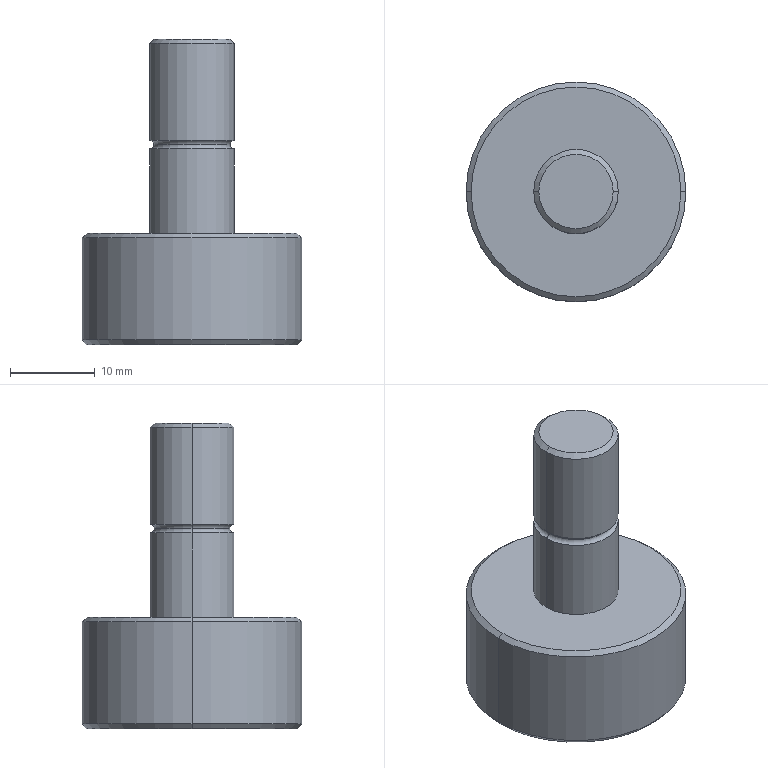Component | SolidWorks | BoltNeedleBearing-1 | 1 solid | 19 faces | box 26 x 26 x 36.2 mm | volume 8774 mm3 | cone 6 | cylinder 6 | torus 4 | plane 3 | commonest cylinder face diameters 10 x4 26 x2
build123d program:
from build123d import *
from OCP.BRepFilletAPI import BRepFilletAPI_MakeChamfer

# Parameters (mm, degrees)
SKETCH1_R           = 13
BOSS_EXTRUDE1_DEPTH = 13.2
SKETCH2_R           = 5
BOSS_EXTRUDE2_DEPTH = 23
CHAMFER1_SIZE       = 0.5
CHAMFER1_SIZE2      = 0.5959
SKETCH3_R           = 0.5
CHAMFER2_SIZE       = 0.5
CHAMFER2_SIZE2      = 0.5959


with BuildPart() as part:
    # Sketch1 → Boss-Extrude1 (new body)
    with BuildSketch(Plane.XY):
        Circle(SKETCH1_R)
    extrude(amount=BOSS_EXTRUDE1_DEPTH)

    # Sketch2 → Boss-Extrude2 (add)
    with BuildSketch(Plane.XY.offset(13.2)):
        Circle(SKETCH2_R)
    extrude(amount=BOSS_EXTRUDE2_DEPTH)

    # Chamfer1
    chamfer1_edges = [part.edges().sort_by_distance(p)[0] for p in [
        (-5, 0, 36.2),
    ]]
    chamfer1_side = [part.faces().sort_by_distance(p)[0] for p in [
        (-5, 0, 24.7),
    ]]
    chamfer(chamfer1_edges, length=CHAMFER1_SIZE, length2=CHAMFER1_SIZE2, reference=chamfer1_side[0])

    # Sketch3 → Cut-Revolve1 (revolve, cut)
    with BuildSketch(Plane(origin=(0, 0, 0), x_dir=(0, 0, -1), z_dir=(1, 0, 0)), mode=Mode.PRIVATE) as cut_revolve1_sk:
        with Locations((-23.7, 5)):
            Circle(SKETCH3_R)
    revolve(cut_revolve1_sk.sketch.rotate(Axis((0, 0, 36.2), (0, 0, -1)), 90), axis=Axis((0, 0, 36.2), (0, 0, -1)), mode=Mode.SUBTRACT)

    # Chamfer2: one chamfer whose edges measure the first distance from different faces: ONE call of the kernel's chamfer builder (chamfer() names one face for all edges)
    chamfer2_edges_1 = [part.edges().sort_by_distance(p)[0] for p in [
        (-13, 0, 0),
    ]]
    chamfer2_side_1 = [part.faces().sort_by_distance(p)[0] for p in [
        (0, 0, 0),
    ]]
    chamfer2_edges_2 = [part.edges().sort_by_distance(p)[0] for p in [
        (-13, 0, 13.2),
    ]]
    chamfer2_side_2 = [part.faces().sort_by_distance(p)[0] for p in [
        (-13, 0, 6.6),
    ]]
    chamfer2 = BRepFilletAPI_MakeChamfer(part.part.solid().wrapped)
    for e in chamfer2_edges_1:
        chamfer2.Add(CHAMFER2_SIZE, CHAMFER2_SIZE2, e.wrapped, chamfer2_side_1[0].wrapped)  # the first distance lies on this face
    for e in chamfer2_edges_2:
        chamfer2.Add(CHAMFER2_SIZE, CHAMFER2_SIZE2, e.wrapped, chamfer2_side_2[0].wrapped)  # the first distance lies on this face
    add(Compound.cast(chamfer2.Shape()), mode=Mode.REPLACE)


solid = part.part

# Placed as in the assembly
solid = solid.moved(Location((-115.847, -83.074, 984.8), (0, 0, 0)))
STEP:
#1=COLOUR_RGB('',0.7922,0.8196,0.9333);
#2=FILL_AREA_STYLE_COLOUR('',#1);
#3=FILL_AREA_STYLE('',(#2));
#4=SURFACE_STYLE_FILL_AREA(#3);
#5=SURFACE_SIDE_STYLE('',(#4));
#6=SURFACE_STYLE_USAGE(.BOTH.,#5);
#7=PRESENTATION_STYLE_ASSIGNMENT((#6));
#8=CARTESIAN_POINT('',(-4.364,-3.271,39.724));
#9=VERTEX_POINT('',#8);
#10=CARTESIAN_POINT('',(-4.384,-3.271,39.705));
#11=VERTEX_POINT('',#10);
#12=CARTESIAN_POINT('',(-4.364,-3.271,39.705));
#13=DIRECTION('',(0.,-1.,-0.));
#14=DIRECTION('',(1.,0.,0.));
#15=AXIS2_PLACEMENT_3D('',#12,#13,#14);
#16=CIRCLE('',#15,0.01969);
#17=EDGE_CURVE('',#9,#11,#16,.T.);
#18=ORIENTED_EDGE('',*,*,#17,.T.);
#19=CARTESIAN_POINT('',(-4.738,-3.271,39.705));
#20=VERTEX_POINT('',#19);
#21=CARTESIAN_POINT('',(-4.561,-3.271,39.705));
#22=DIRECTION('',(0.,-0.,1.));
#23=DIRECTION('',(0.,-1.,0.));
#24=AXIS2_PLACEMENT_3D('',#21,#22,#23);
#25=CIRCLE('',#24,0.1772);
#26=EDGE_CURVE('',#11,#20,#25,.T.);
#27=ORIENTED_EDGE('',*,*,#26,.T.);
#28=CARTESIAN_POINT('',(-4.758,-3.271,39.724));
#29=VERTEX_POINT('',#28);
#30=CARTESIAN_POINT('',(-4.758,-3.271,39.705));
#31=DIRECTION('',(-0.,1.,0.));
#32=DIRECTION('',(-1.,-0.,0.));
#33=AXIS2_PLACEMENT_3D('',#30,#31,#32);
#34=CIRCLE('',#33,0.01969);
#35=EDGE_CURVE('',#29,#20,#34,.T.);
#36=ORIENTED_EDGE('',*,*,#35,.F.);
#37=CARTESIAN_POINT('',(-4.561,-3.271,39.724));
#38=DIRECTION('',(-0.,0.,-1.));
#39=DIRECTION('',(-1.,-0.,0.));
#40=AXIS2_PLACEMENT_3D('',#37,#38,#39);
#41=CIRCLE('',#40,0.1969);
#42=EDGE_CURVE('',#29,#9,#41,.T.);
#43=ORIENTED_EDGE('',*,*,#42,.T.);
#44=EDGE_LOOP('',(#18,#27,#36,#43));
#45=FACE_OUTER_BOUND('',#44,.T.);
#46=CARTESIAN_POINT('',(-4.561,-3.271,39.705));
#47=DIRECTION('',(0.,-0.,1.));
#48=DIRECTION('',(1.,0.,-0.));
#49=AXIS2_PLACEMENT_3D('',#46,#47,#48);
#50=TOROIDAL_SURFACE('',#49,0.1969,0.01969);
#51=ADVANCED_FACE('',(#45),#50,.F.);
#52=ORIENTED_EDGE('',*,*,#35,.T.);
#53=CARTESIAN_POINT('',(-4.561,-3.271,39.705));
#54=DIRECTION('',(0.,-0.,1.));
#55=DIRECTION('',(0.,-1.,0.));
#56=AXIS2_PLACEMENT_3D('',#53,#54,#55);
#57=CIRCLE('',#56,0.1772);
#58=EDGE_CURVE('',#20,#11,#57,.T.);
#59=ORIENTED_EDGE('',*,*,#58,.T.);
#60=ORIENTED_EDGE('',*,*,#17,.F.);
#61=CARTESIAN_POINT('',(-4.561,-3.271,39.724));
#62=DIRECTION('',(-0.,0.,-1.));
#63=DIRECTION('',(-1.,-0.,0.));
#64=AXIS2_PLACEMENT_3D('',#61,#62,#63);
#65=CIRCLE('',#64,0.1969);
#66=EDGE_CURVE('',#9,#29,#65,.T.);
#67=ORIENTED_EDGE('',*,*,#66,.T.);
#68=EDGE_LOOP('',(#52,#59,#60,#67));
#69=FACE_OUTER_BOUND('',#68,.T.);
#70=CARTESIAN_POINT('',(-4.561,-3.271,39.705));
#71=DIRECTION('',(0.,-0.,1.));
#72=DIRECTION('',(1.,0.,-0.));
#73=AXIS2_PLACEMENT_3D('',#70,#71,#72);
#74=TOROIDAL_SURFACE('',#73,0.1969,0.01969);
#75=ADVANCED_FACE('',(#69),#74,.F.);
#76=CARTESIAN_POINT('',(-5.053,-3.271,38.772));
#77=VERTEX_POINT('',#76);
#78=CARTESIAN_POINT('',(-4.069,-3.271,38.772));
#79=VERTEX_POINT('',#78);
#80=CARTESIAN_POINT('',(-4.561,-3.271,38.772));
#81=DIRECTION('',(-0.,0.,-1.));
#82=DIRECTION('',(1.,0.,0.));
#83=AXIS2_PLACEMENT_3D('',#80,#81,#82);
#84=CIRCLE('',#83,0.4921);
#85=EDGE_CURVE('',#77,#79,#84,.T.);
#86=ORIENTED_EDGE('',*,*,#85,.F.);
#87=CARTESIAN_POINT('',(-5.073,-3.271,38.795));
#88=VERTEX_POINT('',#87);
#89=CARTESIAN_POINT('',(-5.073,-3.271,38.795));
#90=DIRECTION('',(-0.6428,-0.,0.766));
#91=VECTOR('',#90,39.37);
#92=LINE('',#89,#91);
#93=EDGE_CURVE('',#77,#88,#92,.T.);
#94=ORIENTED_EDGE('',*,*,#93,.T.);
#95=CARTESIAN_POINT('',(-4.049,-3.271,38.795));
#96=VERTEX_POINT('',#95);
#97=CARTESIAN_POINT('',(-4.561,-3.271,38.795));
#98=DIRECTION('',(0.,-0.,1.));
#99=DIRECTION('',(1.,0.,0.));
#100=AXIS2_PLACEMENT_3D('',#97,#98,#99);
#101=CIRCLE('',#100,0.5118);
#102=EDGE_CURVE('',#96,#88,#101,.T.);
#103=ORIENTED_EDGE('',*,*,#102,.F.);
#104=CARTESIAN_POINT('',(-4.049,-3.271,38.795));
#105=DIRECTION('',(0.6428,0.,0.766));
#106=VECTOR('',#105,39.37);
#107=LINE('',#104,#106);
#108=EDGE_CURVE('',#79,#96,#107,.T.);
#109=ORIENTED_EDGE('',*,*,#108,.F.);
#110=EDGE_LOOP('',(#86,#94,#103,#109));
#111=FACE_OUTER_BOUND('',#110,.T.);
#112=CARTESIAN_POINT('',(-4.561,-3.271,38.795));
#113=DIRECTION('',(0.,-0.,1.));
#114=DIRECTION('',(1.,0.,0.));
#115=AXIS2_PLACEMENT_3D('',#112,#113,#114);
#116=CONICAL_SURFACE('',#115,0.5118,0.6981);
#117=ADVANCED_FACE('',(#111),#116,.T.);
#118=CARTESIAN_POINT('',(-4.073,-3.271,39.291));
#119=VERTEX_POINT('',#118);
#120=CARTESIAN_POINT('',(-5.049,-3.271,39.291));
#121=VERTEX_POINT('',#120);
#122=CARTESIAN_POINT('',(-4.561,-3.271,39.291));
#123=DIRECTION('',(0.,-0.,1.));
#124=DIRECTION('',(1.,0.,0.));
#125=AXIS2_PLACEMENT_3D('',#122,#123,#124);
#126=CIRCLE('',#125,0.4884);
#127=EDGE_CURVE('',#119,#121,#126,.T.);
#128=ORIENTED_EDGE('',*,*,#127,.F.);
#129=CARTESIAN_POINT('',(-4.049,-3.271,39.272));
#130=VERTEX_POINT('',#129);
#131=CARTESIAN_POINT('',(-4.073,-3.271,39.291));
#132=DIRECTION('',(0.766,0.,-0.6428));
#133=VECTOR('',#132,39.37);
#134=LINE('',#131,#133);
#135=EDGE_CURVE('',#119,#130,#134,.T.);
#136=ORIENTED_EDGE('',*,*,#135,.T.);
#137=CARTESIAN_POINT('',(-5.073,-3.271,39.272));
#138=VERTEX_POINT('',#137);
#139=CARTESIAN_POINT('',(-4.561,-3.271,39.272));
#140=DIRECTION('',(-0.,0.,-1.));
#141=DIRECTION('',(1.,0.,0.));
#142=AXIS2_PLACEMENT_3D('',#139,#140,#141);
#143=CIRCLE('',#142,0.5118);
#144=EDGE_CURVE('',#138,#130,#143,.T.);
#145=ORIENTED_EDGE('',*,*,#144,.F.);
#146=CARTESIAN_POINT('',(-5.049,-3.271,39.291));
#147=DIRECTION('',(-0.766,-0.,-0.6428));
#148=VECTOR('',#147,39.37);
#149=LINE('',#146,#148);
#150=EDGE_CURVE('',#121,#138,#149,.T.);
#151=ORIENTED_EDGE('',*,*,#150,.F.);
#152=EDGE_LOOP('',(#128,#136,#145,#151));
#153=FACE_OUTER_BOUND('',#152,.T.);
#154=CARTESIAN_POINT('',(-4.561,-3.271,39.291));
#155=DIRECTION('',(-0.,0.,-1.));
#156=DIRECTION('',(-1.,-0.,0.));
#157=AXIS2_PLACEMENT_3D('',#154,#155,#156);
#158=CONICAL_SURFACE('',#157,0.4884,0.8727);
#159=ADVANCED_FACE('',(#153),#158,.T.);
#160=CARTESIAN_POINT('',(-4.758,-3.271,40.177));
#161=VERTEX_POINT('',#160);
#162=CARTESIAN_POINT('',(-4.364,-3.271,40.177));
#163=VERTEX_POINT('',#162);
#164=CARTESIAN_POINT('',(-4.561,-3.271,40.177));
#165=DIRECTION('',(-0.,0.,-1.));
#166=DIRECTION('',(1.,0.,0.));
#167=AXIS2_PLACEMENT_3D('',#164,#165,#166);
#168=CIRCLE('',#167,0.1969);
#169=EDGE_CURVE('',#161,#163,#168,.T.);
#170=ORIENTED_EDGE('',*,*,#169,.T.);
#171=CARTESIAN_POINT('',(-4.364,-3.271,40.197));
#172=DIRECTION('',(-0.,0.,-1.));
#173=VECTOR('',#172,39.37);
#174=LINE('',#171,#173);
#175=EDGE_CURVE('',#163,#9,#174,.T.);
#176=ORIENTED_EDGE('',*,*,#175,.T.);
#177=ORIENTED_EDGE('',*,*,#42,.F.);
#178=CARTESIAN_POINT('',(-4.758,-3.271,40.197));
#179=DIRECTION('',(-0.,0.,-1.));
#180=VECTOR('',#179,39.37);
#181=LINE('',#178,#180);
#182=EDGE_CURVE('',#161,#29,#181,.T.);
#183=ORIENTED_EDGE('',*,*,#182,.F.);
#184=EDGE_LOOP('',(#170,#176,#177,#183));
#185=FACE_OUTER_BOUND('',#184,.T.);
#186=CARTESIAN_POINT('',(-4.561,-3.271,40.197));
#187=DIRECTION('',(-0.,0.,-1.));
#188=DIRECTION('',(-1.,-0.,0.));
#189=AXIS2_PLACEMENT_3D('',#186,#187,#188);
#190=CYLINDRICAL_SURFACE('',#189,0.1969);
#191=ADVANCED_FACE('',(#185),#190,.T.);
#192=CARTESIAN_POINT('',(-4.388,-3.271,40.197));
#193=VERTEX_POINT('',#192);
#194=CARTESIAN_POINT('',(-4.734,-3.271,40.197));
#195=VERTEX_POINT('',#194);
#196=CARTESIAN_POINT('',(-4.561,-3.271,40.197));
#197=DIRECTION('',(0.,-0.,1.));
#198=DIRECTION('',(1.,0.,0.));
#199=AXIS2_PLACEMENT_3D('',#196,#197,#198);
#200=CIRCLE('',#199,0.1734);
#201=EDGE_CURVE('',#193,#195,#200,.T.);
#202=ORIENTED_EDGE('',*,*,#201,.F.);
#203=CARTESIAN_POINT('',(-4.388,-3.271,40.197));
#204=DIRECTION('',(0.766,0.,-0.6428));
#205=VECTOR('',#204,39.37);
#206=LINE('',#203,#205);
#207=EDGE_CURVE('',#193,#163,#206,.T.);
#208=ORIENTED_EDGE('',*,*,#207,.T.);
#209=ORIENTED_EDGE('',*,*,#169,.F.);
#210=CARTESIAN_POINT('',(-4.734,-3.271,40.197));
#211=DIRECTION('',(-0.766,-0.,-0.6428));
#212=VECTOR('',#211,39.37);
#213=LINE('',#210,#212);
#214=EDGE_CURVE('',#195,#161,#213,.T.);
#215=ORIENTED_EDGE('',*,*,#214,.F.);
#216=EDGE_LOOP('',(#202,#208,#209,#215));
#217=FACE_OUTER_BOUND('',#216,.T.);
#218=CARTESIAN_POINT('',(-4.561,-3.271,40.197));
#219=DIRECTION('',(-0.,0.,-1.));
#220=DIRECTION('',(-1.,-0.,0.));
#221=AXIS2_PLACEMENT_3D('',#218,#219,#220);
#222=CONICAL_SURFACE('',#221,0.1734,0.8727);
#223=ADVANCED_FACE('',(#217),#222,.T.);
#224=ORIENTED_EDGE('',*,*,#58,.F.);
#225=CARTESIAN_POINT('',(-4.758,-3.271,39.685));
#226=VERTEX_POINT('',#225);
#227=CARTESIAN_POINT('',(-4.758,-3.271,39.705));
#228=DIRECTION('',(-0.,1.,0.));
#229=DIRECTION('',(-1.,-0.,0.));
#230=AXIS2_PLACEMENT_3D('',#227,#228,#229);
#231=CIRCLE('',#230,0.01969);
#232=EDGE_CURVE('',#20,#226,#231,.T.);
#233=ORIENTED_EDGE('',*,*,#232,.T.);
#234=CARTESIAN_POINT('',(-4.364,-3.271,39.685));
#235=VERTEX_POINT('',#234);
#236=CARTESIAN_POINT('',(-4.561,-3.271,39.685));
#237=DIRECTION('',(0.,-0.,1.));
#238=DIRECTION('',(1.,0.,0.));
#239=AXIS2_PLACEMENT_3D('',#236,#237,#238);
#240=CIRCLE('',#239,0.1969);
#241=EDGE_CURVE('',#226,#235,#240,.T.);
#242=ORIENTED_EDGE('',*,*,#241,.T.);
#243=CARTESIAN_POINT('',(-4.364,-3.271,39.705));
#244=DIRECTION('',(0.,-1.,-0.));
#245=DIRECTION('',(1.,0.,0.));
#246=AXIS2_PLACEMENT_3D('',#243,#244,#245);
#247=CIRCLE('',#246,0.01969);
#248=EDGE_CURVE('',#11,#235,#247,.T.);
#249=ORIENTED_EDGE('',*,*,#248,.F.);
#250=EDGE_LOOP('',(#224,#233,#242,#249));
#251=FACE_OUTER_BOUND('',#250,.T.);
#252=CARTESIAN_POINT('',(-4.561,-3.271,39.705));
#253=DIRECTION('',(0.,-0.,1.));
#254=DIRECTION('',(1.,0.,-0.));
#255=AXIS2_PLACEMENT_3D('',#252,#253,#254);
#256=TOROIDAL_SURFACE('',#255,0.1969,0.01969);
#257=ADVANCED_FACE('',(#251),#256,.F.);
#258=ORIENTED_EDGE('',*,*,#144,.T.);
#259=CARTESIAN_POINT('',(-4.049,-3.271,39.291));
#260=DIRECTION('',(-0.,0.,-1.));
#261=VECTOR('',#260,39.37);
#262=LINE('',#259,#261);
#263=EDGE_CURVE('',#130,#96,#262,.T.);
#264=ORIENTED_EDGE('',*,*,#263,.T.);
#265=ORIENTED_EDGE('',*,*,#102,.T.);
#266=CARTESIAN_POINT('',(-5.073,-3.271,39.291));
#267=DIRECTION('',(-0.,0.,-1.));
#268=VECTOR('',#267,39.37);
#269=LINE('',#266,#268);
#270=EDGE_CURVE('',#138,#88,#269,.T.);
#271=ORIENTED_EDGE('',*,*,#270,.F.);
#272=EDGE_LOOP('',(#258,#264,#265,#271));
#273=FACE_OUTER_BOUND('',#272,.T.);
#274=CARTESIAN_POINT('',(-4.561,-3.271,39.291));
#275=DIRECTION('',(-0.,0.,-1.));
#276=DIRECTION('',(-1.,-0.,0.));
#277=AXIS2_PLACEMENT_3D('',#274,#275,#276);
#278=CYLINDRICAL_SURFACE('',#277,0.5118);
#279=ADVANCED_FACE('',(#273),#278,.T.);
#280=CARTESIAN_POINT('',(-4.561,-3.271,39.685));
#281=DIRECTION('',(0.,-0.,1.));
#282=DIRECTION('',(1.,0.,0.));
#283=AXIS2_PLACEMENT_3D('',#280,#281,#282);
#284=CIRCLE('',#283,0.1969);
#285=EDGE_CURVE('',#235,#226,#284,.T.);
#286=ORIENTED_EDGE('',*,*,#285,.F.);
#287=CARTESIAN_POINT('',(-4.364,-3.271,39.291));
#288=VERTEX_POINT('',#287);
#289=CARTESIAN_POINT('',(-4.364,-3.271,40.197));
#290=DIRECTION('',(-0.,0.,-1.));
#291=VECTOR('',#290,39.37);
#292=LINE('',#289,#291);
#293=EDGE_CURVE('',#235,#288,#292,.T.);
#294=ORIENTED_EDGE('',*,*,#293,.T.);
#295=CARTESIAN_POINT('',(-4.758,-3.271,39.291));
#296=VERTEX_POINT('',#295);
#297=CARTESIAN_POINT('',(-4.561,-3.271,39.291));
#298=DIRECTION('',(0.,-0.,1.));
#299=DIRECTION('',(1.,0.,0.));
#300=AXIS2_PLACEMENT_3D('',#297,#298,#299);
#301=CIRCLE('',#300,0.1969);
#302=EDGE_CURVE('',#288,#296,#301,.T.);
#303=ORIENTED_EDGE('',*,*,#302,.T.);
#304=CARTESIAN_POINT('',(-4.758,-3.271,40.197));
#305=DIRECTION('',(-0.,0.,-1.));
#306=VECTOR('',#305,39.37);
#307=LINE('',#304,#306);
#308=EDGE_CURVE('',#226,#296,#307,.T.);
#309=ORIENTED_EDGE('',*,*,#308,.F.);
#310=EDGE_LOOP('',(#286,#294,#303,#309));
#311=FACE_OUTER_BOUND('',#310,.T.);
#312=CARTESIAN_POINT('',(-4.561,-3.271,40.197));
#313=DIRECTION('',(-0.,0.,-1.));
#314=DIRECTION('',(-1.,-0.,0.));
#315=AXIS2_PLACEMENT_3D('',#312,#313,#314);
#316=CYLINDRICAL_SURFACE('',#315,0.1969);
#317=ADVANCED_FACE('',(#311),#316,.T.);
#318=ORIENTED_EDGE('',*,*,#293,.F.);
#319=ORIENTED_EDGE('',*,*,#241,.F.);
#320=ORIENTED_EDGE('',*,*,#308,.T.);
#321=CARTESIAN_POINT('',(-4.561,-3.271,39.291));
#322=DIRECTION('',(0.,-0.,1.));
#323=DIRECTION('',(1.,0.,0.));
#324=AXIS2_PLACEMENT_3D('',#321,#322,#323);
#325=CIRCLE('',#324,0.1969);
#326=EDGE_CURVE('',#296,#288,#325,.T.);
#327=ORIENTED_EDGE('',*,*,#326,.T.);
#328=EDGE_LOOP('',(#318,#319,#320,#327));
#329=FACE_OUTER_BOUND('',#328,.T.);
#330=CARTESIAN_POINT('',(-4.561,-3.271,40.197));
#331=DIRECTION('',(-0.,0.,-1.));
#332=DIRECTION('',(-1.,-0.,0.));
#333=AXIS2_PLACEMENT_3D('',#330,#331,#332);
#334=CYLINDRICAL_SURFACE('',#333,0.1969);
#335=ADVANCED_FACE('',(#329),#334,.T.);
#336=ORIENTED_EDGE('',*,*,#263,.F.);
#337=CARTESIAN_POINT('',(-4.561,-3.271,39.272));
#338=DIRECTION('',(-0.,0.,-1.));
#339=DIRECTION('',(1.,0.,0.));
#340=AXIS2_PLACEMENT_3D('',#337,#338,#339);
#341=CIRCLE('',#340,0.5118);
#342=EDGE_CURVE('',#130,#138,#341,.T.);
#343=ORIENTED_EDGE('',*,*,#342,.T.);
#344=ORIENTED_EDGE('',*,*,#270,.T.);
#345=CARTESIAN_POINT('',(-4.561,-3.271,38.795));
#346=DIRECTION('',(0.,-0.,1.));
#347=DIRECTION('',(1.,0.,0.));
#348=AXIS2_PLACEMENT_3D('',#345,#346,#347);
#349=CIRCLE('',#348,0.5118);
#350=EDGE_CURVE('',#88,#96,#349,.T.);
#351=ORIENTED_EDGE('',*,*,#350,.T.);
#352=EDGE_LOOP('',(#336,#343,#344,#351));
#353=FACE_OUTER_BOUND('',#352,.T.);
#354=CARTESIAN_POINT('',(-4.561,-3.271,39.291));
#355=DIRECTION('',(-0.,0.,-1.));
#356=DIRECTION('',(-1.,-0.,0.));
#357=AXIS2_PLACEMENT_3D('',#354,#355,#356);
#358=CYLINDRICAL_SURFACE('',#357,0.5118);
#359=ADVANCED_FACE('',(#353),#358,.T.);
#360=CARTESIAN_POINT('',(-4.561,-3.271,39.291));
#361=DIRECTION('',(0.,-0.,1.));
#362=DIRECTION('',(1.,0.,0.));
#363=AXIS2_PLACEMENT_3D('',#360,#361,#362);
#364=CIRCLE('',#363,0.4884);
#365=EDGE_CURVE('',#121,#119,#364,.T.);
#366=ORIENTED_EDGE('',*,*,#365,.T.);
#367=ORIENTED_EDGE('',*,*,#127,.T.);
#368=EDGE_LOOP('',(#366,#367));
#369=FACE_OUTER_BOUND('',#368,.T.);
#370=ORIENTED_EDGE('',*,*,#326,.F.);
#371=ORIENTED_EDGE('',*,*,#302,.F.);
#372=EDGE_LOOP('',(#370,#371));
#373=FACE_BOUND('',#372,.T.);
#374=CARTESIAN_POINT('',(-4.561,-3.271,39.291));
#375=DIRECTION('',(0.,-0.,1.));
#376=DIRECTION('',(1.,0.,-0.));
#377=AXIS2_PLACEMENT_3D('',#374,#375,#376);
#378=PLANE('',#377);
#379=ADVANCED_FACE('',(#369,#373),#378,.T.);
#380=CARTESIAN_POINT('',(-4.561,-3.271,38.772));
#381=DIRECTION('',(-0.,0.,-1.));
#382=DIRECTION('',(1.,0.,0.));
#383=AXIS2_PLACEMENT_3D('',#380,#381,#382);
#384=CIRCLE('',#383,0.4921);
#385=EDGE_CURVE('',#79,#77,#384,.T.);
#386=ORIENTED_EDGE('',*,*,#385,.T.);
#387=ORIENTED_EDGE('',*,*,#85,.T.);
#388=EDGE_LOOP('',(#386,#387));
#389=FACE_OUTER_BOUND('',#388,.T.);
#390=CARTESIAN_POINT('',(-4.561,-3.271,38.772));
#391=DIRECTION('',(0.,-0.,1.));
#392=DIRECTION('',(1.,0.,-0.));
#393=AXIS2_PLACEMENT_3D('',#390,#391,#392);
#394=PLANE('',#393);
#395=ADVANCED_FACE('',(#389),#394,.F.);
#396=ORIENTED_EDGE('',*,*,#26,.F.);
#397=ORIENTED_EDGE('',*,*,#248,.T.);
#398=ORIENTED_EDGE('',*,*,#285,.T.);
#399=ORIENTED_EDGE('',*,*,#232,.F.);
#400=EDGE_LOOP('',(#396,#397,#398,#399));
#401=FACE_OUTER_BOUND('',#400,.T.);
#402=CARTESIAN_POINT('',(-4.561,-3.271,39.705));
#403=DIRECTION('',(0.,-0.,1.));
#404=DIRECTION('',(1.,0.,-0.));
#405=AXIS2_PLACEMENT_3D('',#402,#403,#404);
#406=TOROIDAL_SURFACE('',#405,0.1969,0.01969);
#407=ADVANCED_FACE('',(#401),#406,.F.);
#408=CARTESIAN_POINT('',(-4.561,-3.271,40.197));
#409=DIRECTION('',(0.,-0.,1.));
#410=DIRECTION('',(1.,0.,0.));
#411=AXIS2_PLACEMENT_3D('',#408,#409,#410);
#412=CIRCLE('',#411,0.1734);
#413=EDGE_CURVE('',#195,#193,#412,.T.);
#414=ORIENTED_EDGE('',*,*,#413,.T.);
#415=ORIENTED_EDGE('',*,*,#201,.T.);
#416=EDGE_LOOP('',(#414,#415));
#417=FACE_OUTER_BOUND('',#416,.T.);
#418=CARTESIAN_POINT('',(-4.561,-3.271,40.197));
#419=DIRECTION('',(0.,-0.,1.));
#420=DIRECTION('',(1.,0.,-0.));
#421=AXIS2_PLACEMENT_3D('',#418,#419,#420);
#422=PLANE('',#421);
#423=ADVANCED_FACE('',(#417),#422,.T.);
#424=ORIENTED_EDGE('',*,*,#207,.F.);
#425=ORIENTED_EDGE('',*,*,#413,.F.);
#426=ORIENTED_EDGE('',*,*,#214,.T.);
#427=CARTESIAN_POINT('',(-4.561,-3.271,40.177));
#428=DIRECTION('',(-0.,0.,-1.));
#429=DIRECTION('',(1.,0.,0.));
#430=AXIS2_PLACEMENT_3D('',#427,#428,#429);
#431=CIRCLE('',#430,0.1969);
#432=EDGE_CURVE('',#163,#161,#431,.T.);
#433=ORIENTED_EDGE('',*,*,#432,.F.);
#434=EDGE_LOOP('',(#424,#425,#426,#433));
#435=FACE_OUTER_BOUND('',#434,.T.);
#436=CARTESIAN_POINT('',(-4.561,-3.271,40.197));
#437=DIRECTION('',(-0.,0.,-1.));
#438=DIRECTION('',(-1.,-0.,0.));
#439=AXIS2_PLACEMENT_3D('',#436,#437,#438);
#440=CONICAL_SURFACE('',#439,0.1734,0.8727);
#441=ADVANCED_FACE('',(#435),#440,.T.);
#442=ORIENTED_EDGE('',*,*,#175,.F.);
#443=ORIENTED_EDGE('',*,*,#432,.T.);
#444=ORIENTED_EDGE('',*,*,#182,.T.);
#445=ORIENTED_EDGE('',*,*,#66,.F.);
#446=EDGE_LOOP('',(#442,#443,#444,#445));
#447=FACE_OUTER_BOUND('',#446,.T.);
#448=CARTESIAN_POINT('',(-4.561,-3.271,40.197));
#449=DIRECTION('',(-0.,0.,-1.));
#450=DIRECTION('',(-1.,-0.,0.));
#451=AXIS2_PLACEMENT_3D('',#448,#449,#450);
#452=CYLINDRICAL_SURFACE('',#451,0.1969);
#453=ADVANCED_FACE('',(#447),#452,.T.);
#454=ORIENTED_EDGE('',*,*,#135,.F.);
#455=ORIENTED_EDGE('',*,*,#365,.F.);
#456=ORIENTED_EDGE('',*,*,#150,.T.);
#457=ORIENTED_EDGE('',*,*,#342,.F.);
#458=EDGE_LOOP('',(#454,#455,#456,#457));
#459=FACE_OUTER_BOUND('',#458,.T.);
#460=CARTESIAN_POINT('',(-4.561,-3.271,39.291));
#461=DIRECTION('',(-0.,0.,-1.));
#462=DIRECTION('',(-1.,-0.,0.));
#463=AXIS2_PLACEMENT_3D('',#460,#461,#462);
#464=CONICAL_SURFACE('',#463,0.4884,0.8727);
#465=ADVANCED_FACE('',(#459),#464,.T.);
#466=ORIENTED_EDGE('',*,*,#93,.F.);
#467=ORIENTED_EDGE('',*,*,#385,.F.);
#468=ORIENTED_EDGE('',*,*,#108,.T.);
#469=ORIENTED_EDGE('',*,*,#350,.F.);
#470=EDGE_LOOP('',(#466,#467,#468,#469));
#471=FACE_OUTER_BOUND('',#470,.T.);
#472=CARTESIAN_POINT('',(-4.561,-3.271,38.795));
#473=DIRECTION('',(0.,-0.,1.));
#474=DIRECTION('',(1.,0.,0.));
#475=AXIS2_PLACEMENT_3D('',#472,#473,#474);
#476=CONICAL_SURFACE('',#475,0.5118,0.6981);
#477=ADVANCED_FACE('',(#471),#476,.T.);
#478=CLOSED_SHELL('',(#51,#75,#117,#159,#191,#223,#257,#279,#317,#335,#359,#379,#395,#407,#423,#441,#453,#465,#477));
#479=MANIFOLD_SOLID_BREP('',#478);
#480=STYLED_ITEM('',(#7),#479);
#481=PRESENTATION_LAYER_ASSIGNMENT('','',(#480));
#482=CARTESIAN_POINT('',(0.,0.,0.));
#483=DIRECTION('',(0.,0.,1.));
#484=DIRECTION('',(1.,0.,0.));
#485=AXIS2_PLACEMENT_3D('',#482,#483,#484);
#486=(LENGTH_UNIT()NAMED_UNIT(*)SI_UNIT($,.METRE.));
#487=LENGTH_MEASURE_WITH_UNIT(LENGTH_MEASURE(0.0254),#486);
#488=DIMENSIONAL_EXPONENTS(1.,0.,0.,0.,0.,0.,0.);
#489=(CONVERSION_BASED_UNIT('',#487)LENGTH_UNIT()NAMED_UNIT(#488));
#490=UNCERTAINTY_MEASURE_WITH_UNIT(LENGTH_MEASURE(0.00001),#489,'','');
#491=(NAMED_UNIT(*)PLANE_ANGLE_UNIT()SI_UNIT($,.RADIAN.));
#492=(NAMED_UNIT(*)SI_UNIT($,.STERADIAN.)SOLID_ANGLE_UNIT());
#493=(GEOMETRIC_REPRESENTATION_CONTEXT(3)GLOBAL_UNCERTAINTY_ASSIGNED_CONTEXT((#490))GLOBAL_UNIT_ASSIGNED_CONTEXT((#489,#491,#492))REPRESENTATION_CONTEXT('',''));
#494=ADVANCED_BREP_SHAPE_REPRESENTATION('',(#479,#485),#493);
#495=(LENGTH_UNIT()NAMED_UNIT(*)SI_UNIT($,.METRE.));
#496=LENGTH_MEASURE_WITH_UNIT(LENGTH_MEASURE(0.0254),#495);
#497=DIMENSIONAL_EXPONENTS(1.,0.,0.,0.,0.,0.,0.);
#498=(CONVERSION_BASED_UNIT('',#496)LENGTH_UNIT()NAMED_UNIT(#497));
#499=UNCERTAINTY_MEASURE_WITH_UNIT(LENGTH_MEASURE(0.00001),#498,'','');
#500=(NAMED_UNIT(*)PLANE_ANGLE_UNIT()SI_UNIT($,.RADIAN.));
#501=(NAMED_UNIT(*)SI_UNIT($,.STERADIAN.)SOLID_ANGLE_UNIT());
#502=(GEOMETRIC_REPRESENTATION_CONTEXT(3)GLOBAL_UNCERTAINTY_ASSIGNED_CONTEXT((#499))GLOBAL_UNIT_ASSIGNED_CONTEXT((#498,#500,#501))REPRESENTATION_CONTEXT('',''));
#503=MECHANICAL_DESIGN_GEOMETRIC_PRESENTATION_REPRESENTATION('',(#480),#502);